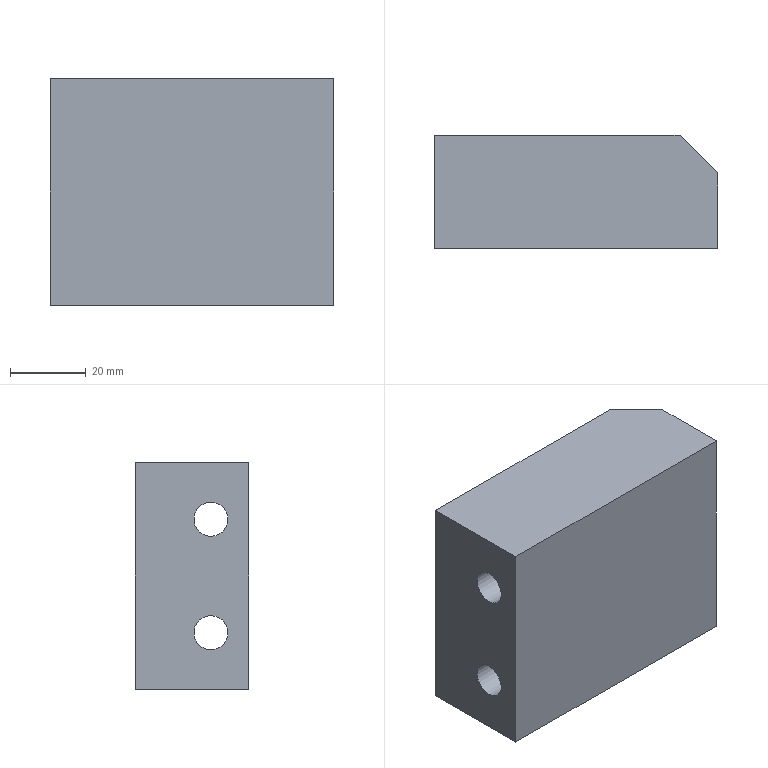Component | NX | BLOCK | 1 solid | 13 faces | box 75 x 30 x 60 mm | volume 109112 mm3 | plane 9 | cylinder 4 | commonest cylinder face diameters 9 x2 15 x2
STEP:
#1=CARTESIAN_POINT('',(0.,0.,0.));
#2=DIRECTION('',(0.,0.,1.));
#3=DIRECTION('',(1.,0.,0.));
#4=AXIS2_PLACEMENT_3D('',#1,#2,#3);
#5=CARTESIAN_POINT('',(2.092,116.121,56.345));
#6=VERTEX_POINT('',#5);
#7=CARTESIAN_POINT('',(2.092,116.121,48.845));
#8=DIRECTION('',(-1.,0.,0.));
#9=DIRECTION('',(0.,0.,1.));
#10=AXIS2_PLACEMENT_3D('',#7,#8,#9);
#11=CIRCLE('',#10,7.5);
#12=CARTESIAN_POINT('',(2.092,121.121,63.845));
#13=DIRECTION('',(1.,0.,0.));
#14=DIRECTION('',(0.,0.,-1.));
#15=AXIS2_PLACEMENT_3D('',#12,#13,#14);
#16=PLANE('',#15);
#17=CARTESIAN_POINT('',(7.5,-5.));
#18=CARTESIAN_POINT('',(7.5,7.99));
#19=CARTESIAN_POINT('',(18.75,1.495));
#20=CARTESIAN_POINT('',(30.,-5.));
#21=CARTESIAN_POINT('',(18.75,-11.495));
#22=CARTESIAN_POINT('',(7.5,-17.99));
#23=CARTESIAN_POINT('',(7.5,-5.));
#24=(BOUNDED_CURVE()B_SPLINE_CURVE(2,(#17,#18,#19,#20,#21,#22,#23),.UNSPECIFIED.,.T.,.F.)B_SPLINE_CURVE_WITH_KNOTS((1,2,2,2,2,1),(-2.094,0.,2.094,4.189,6.283,8.378),.UNSPECIFIED.)CURVE()GEOMETRIC_REPRESENTATION_ITEM()RATIONAL_B_SPLINE_CURVE((1.,0.5,1.,0.5,1.,0.5,1.))REPRESENTATION_ITEM(''));
#25=(GEOMETRIC_REPRESENTATION_CONTEXT(2)PARAMETRIC_REPRESENTATION_CONTEXT()REPRESENTATION_CONTEXT('',''));
#26=DEFINITIONAL_REPRESENTATION('',(#24),#25);
#27=PCURVE('',#16,#26);
#28=CARTESIAN_POINT('',(2.092,116.121,48.845));
#29=DIRECTION('',(-1.,0.,0.));
#30=DIRECTION('',(0.,0.,1.));
#31=AXIS2_PLACEMENT_3D('',#28,#29,#30);
#32=CYLINDRICAL_SURFACE('',#31,7.5);
#33=CARTESIAN_POINT('',(0.,0.));
#34=DIRECTION('',(1.,0.));
#35=VECTOR('',#34,1.);
#36=LINE('',#33,#35);
#37=(GEOMETRIC_REPRESENTATION_CONTEXT(2)PARAMETRIC_REPRESENTATION_CONTEXT()REPRESENTATION_CONTEXT('',''));
#38=DEFINITIONAL_REPRESENTATION('',(#36),#37);
#39=PCURVE('',#32,#38);
#40=SURFACE_CURVE('',#11,(#27,#39),.PCURVE_S1.);
#41=EDGE_CURVE('',#6,#6,#40,.T.);
#42=ORIENTED_EDGE('',*,*,#41,.T.);
#43=EDGE_LOOP('',(#42));
#44=FACE_BOUND('',#43,.T.);
#45=CARTESIAN_POINT('',(2.092,116.121,86.345));
#46=VERTEX_POINT('',#45);
#47=CARTESIAN_POINT('',(2.092,116.121,78.845));
#48=DIRECTION('',(-1.,0.,0.));
#49=DIRECTION('',(0.,0.,1.));
#50=AXIS2_PLACEMENT_3D('',#47,#48,#49);
#51=CIRCLE('',#50,7.5);
#52=CARTESIAN_POINT('',(-22.5,-5.));
#53=CARTESIAN_POINT('',(-22.5,7.99));
#54=CARTESIAN_POINT('',(-11.25,1.495));
#55=CARTESIAN_POINT('',(-0.,-5.));
#56=CARTESIAN_POINT('',(-11.25,-11.495));
#57=CARTESIAN_POINT('',(-22.5,-17.99));
#58=CARTESIAN_POINT('',(-22.5,-5.));
#59=(BOUNDED_CURVE()B_SPLINE_CURVE(2,(#52,#53,#54,#55,#56,#57,#58),.UNSPECIFIED.,.T.,.F.)B_SPLINE_CURVE_WITH_KNOTS((1,2,2,2,2,1),(-2.094,0.,2.094,4.189,6.283,8.378),.UNSPECIFIED.)CURVE()GEOMETRIC_REPRESENTATION_ITEM()RATIONAL_B_SPLINE_CURVE((1.,0.5,1.,0.5,1.,0.5,1.))REPRESENTATION_ITEM(''));
#60=(GEOMETRIC_REPRESENTATION_CONTEXT(2)PARAMETRIC_REPRESENTATION_CONTEXT()REPRESENTATION_CONTEXT('',''));
#61=DEFINITIONAL_REPRESENTATION('',(#59),#60);
#62=PCURVE('',#16,#61);
#63=CARTESIAN_POINT('',(2.092,116.121,78.845));
#64=DIRECTION('',(-1.,0.,0.));
#65=DIRECTION('',(0.,0.,1.));
#66=AXIS2_PLACEMENT_3D('',#63,#64,#65);
#67=CYLINDRICAL_SURFACE('',#66,7.5);
#68=CARTESIAN_POINT('',(0.,0.));
#69=DIRECTION('',(1.,0.));
#70=VECTOR('',#69,1.);
#71=LINE('',#68,#70);
#72=(GEOMETRIC_REPRESENTATION_CONTEXT(2)PARAMETRIC_REPRESENTATION_CONTEXT()REPRESENTATION_CONTEXT('',''));
#73=DEFINITIONAL_REPRESENTATION('',(#71),#72);
#74=PCURVE('',#67,#73);
#75=SURFACE_CURVE('',#51,(#62,#74),.PCURVE_S1.);
#76=EDGE_CURVE('',#46,#46,#75,.T.);
#77=ORIENTED_EDGE('',*,*,#76,.T.);
#78=EDGE_LOOP('',(#77));
#79=FACE_BOUND('',#78,.T.);
#80=CARTESIAN_POINT('',(2.092,126.121,33.845));
#81=VERTEX_POINT('',#80);
#82=CARTESIAN_POINT('',(2.092,106.121,33.845));
#83=VERTEX_POINT('',#82);
#84=CARTESIAN_POINT('',(2.092,121.121,33.845));
#85=DIRECTION('',(0.,-1.,0.));
#86=VECTOR('',#85,1.);
#87=LINE('',#84,#86);
#88=CARTESIAN_POINT('',(30.,0.));
#89=DIRECTION('',(0.,-1.));
#90=VECTOR('',#89,1.);
#91=LINE('',#88,#90);
#92=(GEOMETRIC_REPRESENTATION_CONTEXT(2)PARAMETRIC_REPRESENTATION_CONTEXT()REPRESENTATION_CONTEXT('',''));
#93=DEFINITIONAL_REPRESENTATION('',(#91),#92);
#94=PCURVE('',#16,#93);
#95=CARTESIAN_POINT('',(-72.908,121.121,33.845));
#96=DIRECTION('',(0.,0.,-1.));
#97=DIRECTION('',(-1.,0.,0.));
#98=AXIS2_PLACEMENT_3D('',#95,#96,#97);
#99=PLANE('',#98);
#100=CARTESIAN_POINT('',(-75.,0.));
#101=DIRECTION('',(0.,-1.));
#102=VECTOR('',#101,1.);
#103=LINE('',#100,#102);
#104=(GEOMETRIC_REPRESENTATION_CONTEXT(2)PARAMETRIC_REPRESENTATION_CONTEXT()REPRESENTATION_CONTEXT('',''));
#105=DEFINITIONAL_REPRESENTATION('',(#103),#104);
#106=PCURVE('',#99,#105);
#107=SURFACE_CURVE('',#87,(#94,#106),.PCURVE_S1.);
#108=EDGE_CURVE('',#81,#83,#107,.T.);
#109=ORIENTED_EDGE('',*,*,#108,.F.);
#110=CARTESIAN_POINT('',(2.092,126.121,93.845));
#111=VERTEX_POINT('',#110);
#112=CARTESIAN_POINT('',(2.092,126.121,63.845));
#113=DIRECTION('',(0.,0.,1.));
#114=VECTOR('',#113,1.);
#115=LINE('',#112,#114);
#116=CARTESIAN_POINT('',(0.,5.));
#117=DIRECTION('',(-1.,0.));
#118=VECTOR('',#117,1.);
#119=LINE('',#116,#118);
#120=(GEOMETRIC_REPRESENTATION_CONTEXT(2)PARAMETRIC_REPRESENTATION_CONTEXT()REPRESENTATION_CONTEXT('',''));
#121=DEFINITIONAL_REPRESENTATION('',(#119),#120);
#122=PCURVE('',#16,#121);
#123=CARTESIAN_POINT('',(-7.908,136.121,63.845));
#124=DIRECTION('',(-0.7071,-0.7071,0.));
#125=DIRECTION('',(0.,0.,-1.));
#126=AXIS2_PLACEMENT_3D('',#123,#124,#125);
#127=PLANE('',#126);
#128=CARTESIAN_POINT('',(0.,14.142));
#129=DIRECTION('',(-1.,0.));
#130=VECTOR('',#129,1.);
#131=LINE('',#128,#130);
#132=(GEOMETRIC_REPRESENTATION_CONTEXT(2)PARAMETRIC_REPRESENTATION_CONTEXT()REPRESENTATION_CONTEXT('',''));
#133=DEFINITIONAL_REPRESENTATION('',(#131),#132);
#134=PCURVE('',#127,#133);
#135=SURFACE_CURVE('',#115,(#122,#134),.PCURVE_S1.);
#136=EDGE_CURVE('',#81,#111,#135,.T.);
#137=ORIENTED_EDGE('',*,*,#136,.T.);
#138=CARTESIAN_POINT('',(2.092,106.121,93.845));
#139=VERTEX_POINT('',#138);
#140=CARTESIAN_POINT('',(2.092,121.121,93.845));
#141=DIRECTION('',(0.,1.,0.));
#142=VECTOR('',#141,1.);
#143=LINE('',#140,#142);
#144=CARTESIAN_POINT('',(-30.,0.));
#145=DIRECTION('',(0.,1.));
#146=VECTOR('',#145,1.);
#147=LINE('',#144,#146);
#148=(GEOMETRIC_REPRESENTATION_CONTEXT(2)PARAMETRIC_REPRESENTATION_CONTEXT()REPRESENTATION_CONTEXT('',''));
#149=DEFINITIONAL_REPRESENTATION('',(#147),#148);
#150=PCURVE('',#16,#149);
#151=CARTESIAN_POINT('',(-72.908,121.121,93.845));
#152=DIRECTION('',(0.,0.,1.));
#153=DIRECTION('',(1.,0.,0.));
#154=AXIS2_PLACEMENT_3D('',#151,#152,#153);
#155=PLANE('',#154);
#156=CARTESIAN_POINT('',(75.,0.));
#157=DIRECTION('',(0.,1.));
#158=VECTOR('',#157,1.);
#159=LINE('',#156,#158);
#160=(GEOMETRIC_REPRESENTATION_CONTEXT(2)PARAMETRIC_REPRESENTATION_CONTEXT()REPRESENTATION_CONTEXT('',''));
#161=DEFINITIONAL_REPRESENTATION('',(#159),#160);
#162=PCURVE('',#155,#161);
#163=SURFACE_CURVE('',#143,(#150,#162),.PCURVE_S1.);
#164=EDGE_CURVE('',#139,#111,#163,.T.);
#165=ORIENTED_EDGE('',*,*,#164,.F.);
#166=CARTESIAN_POINT('',(2.092,106.121,63.845));
#167=DIRECTION('',(0.,0.,1.));
#168=VECTOR('',#167,1.);
#169=LINE('',#166,#168);
#170=CARTESIAN_POINT('',(0.,-15.));
#171=DIRECTION('',(-1.,0.));
#172=VECTOR('',#171,1.);
#173=LINE('',#170,#172);
#174=(GEOMETRIC_REPRESENTATION_CONTEXT(2)PARAMETRIC_REPRESENTATION_CONTEXT()REPRESENTATION_CONTEXT('',''));
#175=DEFINITIONAL_REPRESENTATION('',(#173),#174);
#176=PCURVE('',#16,#175);
#177=CARTESIAN_POINT('',(-72.908,106.121,63.845));
#178=DIRECTION('',(0.,-1.,0.));
#179=DIRECTION('',(-1.,0.,0.));
#180=AXIS2_PLACEMENT_3D('',#177,#178,#179);
#181=PLANE('',#180);
#182=CARTESIAN_POINT('',(-75.,0.));
#183=DIRECTION('',(0.,-1.));
#184=VECTOR('',#183,1.);
#185=LINE('',#182,#184);
#186=(GEOMETRIC_REPRESENTATION_CONTEXT(2)PARAMETRIC_REPRESENTATION_CONTEXT()REPRESENTATION_CONTEXT('',''));
#187=DEFINITIONAL_REPRESENTATION('',(#185),#186);
#188=PCURVE('',#181,#187);
#189=SURFACE_CURVE('',#169,(#176,#188),.PCURVE_S1.);
#190=EDGE_CURVE('',#83,#139,#189,.T.);
#191=ORIENTED_EDGE('',*,*,#190,.F.);
#192=EDGE_LOOP('',(#109,#137,#165,#191));
#193=FACE_BOUND('',#192,.T.);
#194=ADVANCED_FACE('',(#44,#79,#193),#16,.T.);
#195=CARTESIAN_POINT('',(-72.908,106.121,33.845));
#196=VERTEX_POINT('',#195);
#197=CARTESIAN_POINT('',(-72.908,106.121,33.845));
#198=DIRECTION('',(1.,0.,0.));
#199=VECTOR('',#198,1.);
#200=LINE('',#197,#199);
#201=CARTESIAN_POINT('',(0.,30.));
#202=DIRECTION('',(-1.,0.));
#203=VECTOR('',#202,1.);
#204=LINE('',#201,#203);
#205=(GEOMETRIC_REPRESENTATION_CONTEXT(2)PARAMETRIC_REPRESENTATION_CONTEXT()REPRESENTATION_CONTEXT('',''));
#206=DEFINITIONAL_REPRESENTATION('',(#204),#205);
#207=PCURVE('',#181,#206);
#208=CARTESIAN_POINT('',(0.,-15.));
#209=DIRECTION('',(-1.,0.));
#210=VECTOR('',#209,1.);
#211=LINE('',#208,#210);
#212=(GEOMETRIC_REPRESENTATION_CONTEXT(2)PARAMETRIC_REPRESENTATION_CONTEXT()REPRESENTATION_CONTEXT('',''));
#213=DEFINITIONAL_REPRESENTATION('',(#211),#212);
#214=PCURVE('',#99,#213);
#215=SURFACE_CURVE('',#200,(#207,#214),.PCURVE_S1.);
#216=EDGE_CURVE('',#196,#83,#215,.T.);
#217=ORIENTED_EDGE('',*,*,#216,.T.);
#218=ORIENTED_EDGE('',*,*,#190,.T.);
#219=CARTESIAN_POINT('',(-72.908,106.121,93.845));
#220=VERTEX_POINT('',#219);
#221=CARTESIAN_POINT('',(-72.908,106.121,93.845));
#222=DIRECTION('',(1.,0.,0.));
#223=VECTOR('',#222,1.);
#224=LINE('',#221,#223);
#225=CARTESIAN_POINT('',(0.,-30.));
#226=DIRECTION('',(-1.,0.));
#227=VECTOR('',#226,1.);
#228=LINE('',#225,#227);
#229=(GEOMETRIC_REPRESENTATION_CONTEXT(2)PARAMETRIC_REPRESENTATION_CONTEXT()REPRESENTATION_CONTEXT('',''));
#230=DEFINITIONAL_REPRESENTATION('',(#228),#229);
#231=PCURVE('',#181,#230);
#232=CARTESIAN_POINT('',(0.,-15.));
#233=DIRECTION('',(1.,0.));
#234=VECTOR('',#233,1.);
#235=LINE('',#232,#234);
#236=(GEOMETRIC_REPRESENTATION_CONTEXT(2)PARAMETRIC_REPRESENTATION_CONTEXT()REPRESENTATION_CONTEXT('',''));
#237=DEFINITIONAL_REPRESENTATION('',(#235),#236);
#238=PCURVE('',#155,#237);
#239=SURFACE_CURVE('',#224,(#231,#238),.PCURVE_S1.);
#240=EDGE_CURVE('',#220,#139,#239,.T.);
#241=ORIENTED_EDGE('',*,*,#240,.F.);
#242=CARTESIAN_POINT('',(-72.908,106.121,63.845));
#243=DIRECTION('',(0.,0.,-1.));
#244=VECTOR('',#243,1.);
#245=LINE('',#242,#244);
#246=CARTESIAN_POINT('',(0.,0.));
#247=DIRECTION('',(0.,1.));
#248=VECTOR('',#247,1.);
#249=LINE('',#246,#248);
#250=(GEOMETRIC_REPRESENTATION_CONTEXT(2)PARAMETRIC_REPRESENTATION_CONTEXT()REPRESENTATION_CONTEXT('',''));
#251=DEFINITIONAL_REPRESENTATION('',(#249),#250);
#252=PCURVE('',#181,#251);
#253=CARTESIAN_POINT('',(-72.908,121.121,63.845));
#254=DIRECTION('',(-1.,0.,0.));
#255=DIRECTION('',(0.,0.,1.));
#256=AXIS2_PLACEMENT_3D('',#253,#254,#255);
#257=PLANE('',#256);
#258=CARTESIAN_POINT('',(0.,-15.));
#259=DIRECTION('',(-1.,0.));
#260=VECTOR('',#259,1.);
#261=LINE('',#258,#260);
#262=(GEOMETRIC_REPRESENTATION_CONTEXT(2)PARAMETRIC_REPRESENTATION_CONTEXT()REPRESENTATION_CONTEXT('',''));
#263=DEFINITIONAL_REPRESENTATION('',(#261),#262);
#264=PCURVE('',#257,#263);
#265=SURFACE_CURVE('',#245,(#252,#264),.PCURVE_S1.);
#266=EDGE_CURVE('',#220,#196,#265,.T.);
#267=ORIENTED_EDGE('',*,*,#266,.T.);
#268=EDGE_LOOP('',(#217,#218,#241,#267));
#269=FACE_BOUND('',#268,.T.);
#270=ADVANCED_FACE('',(#269),#181,.T.);
#271=ORIENTED_EDGE('',*,*,#164,.T.);
#272=CARTESIAN_POINT('',(-7.908,136.121,93.845));
#273=VERTEX_POINT('',#272);
#274=CARTESIAN_POINT('',(-32.908,161.121,93.845));
#275=DIRECTION('',(-0.7071,0.7071,0.));
#276=VECTOR('',#275,1.);
#277=LINE('',#274,#276);
#278=CARTESIAN_POINT('',(40.,40.));
#279=DIRECTION('',(-0.7071,0.7071));
#280=VECTOR('',#279,1.);
#281=LINE('',#278,#280);
#282=(GEOMETRIC_REPRESENTATION_CONTEXT(2)PARAMETRIC_REPRESENTATION_CONTEXT()REPRESENTATION_CONTEXT('',''));
#283=DEFINITIONAL_REPRESENTATION('',(#281),#282);
#284=PCURVE('',#155,#283);
#285=CARTESIAN_POINT('',(-30.,-35.355));
#286=DIRECTION('',(0.,-1.));
#287=VECTOR('',#286,1.);
#288=LINE('',#285,#287);
#289=(GEOMETRIC_REPRESENTATION_CONTEXT(2)PARAMETRIC_REPRESENTATION_CONTEXT()REPRESENTATION_CONTEXT('',''));
#290=DEFINITIONAL_REPRESENTATION('',(#288),#289);
#291=PCURVE('',#127,#290);
#292=SURFACE_CURVE('',#277,(#284,#291),.PCURVE_S1.);
#293=EDGE_CURVE('',#111,#273,#292,.T.);
#294=ORIENTED_EDGE('',*,*,#293,.T.);
#295=CARTESIAN_POINT('',(-72.908,136.121,93.845));
#296=VERTEX_POINT('',#295);
#297=CARTESIAN_POINT('',(-72.908,136.121,93.845));
#298=DIRECTION('',(1.,0.,0.));
#299=VECTOR('',#298,1.);
#300=LINE('',#297,#299);
#301=CARTESIAN_POINT('',(0.,15.));
#302=DIRECTION('',(1.,0.));
#303=VECTOR('',#302,1.);
#304=LINE('',#301,#303);
#305=(GEOMETRIC_REPRESENTATION_CONTEXT(2)PARAMETRIC_REPRESENTATION_CONTEXT()REPRESENTATION_CONTEXT('',''));
#306=DEFINITIONAL_REPRESENTATION('',(#304),#305);
#307=PCURVE('',#155,#306);
#308=CARTESIAN_POINT('',(-72.908,136.121,63.845));
#309=DIRECTION('',(0.,1.,0.));
#310=DIRECTION('',(1.,0.,0.));
#311=AXIS2_PLACEMENT_3D('',#308,#309,#310);
#312=PLANE('',#311);
#313=CARTESIAN_POINT('',(0.,-30.));
#314=DIRECTION('',(1.,0.));
#315=VECTOR('',#314,1.);
#316=LINE('',#313,#315);
#317=(GEOMETRIC_REPRESENTATION_CONTEXT(2)PARAMETRIC_REPRESENTATION_CONTEXT()REPRESENTATION_CONTEXT('',''));
#318=DEFINITIONAL_REPRESENTATION('',(#316),#317);
#319=PCURVE('',#312,#318);
#320=SURFACE_CURVE('',#300,(#307,#319),.PCURVE_S1.);
#321=EDGE_CURVE('',#296,#273,#320,.T.);
#322=ORIENTED_EDGE('',*,*,#321,.F.);
#323=CARTESIAN_POINT('',(-72.908,121.121,93.845));
#324=DIRECTION('',(0.,-1.,0.));
#325=VECTOR('',#324,1.);
#326=LINE('',#323,#325);
#327=CARTESIAN_POINT('',(0.,0.));
#328=DIRECTION('',(0.,-1.));
#329=VECTOR('',#328,1.);
#330=LINE('',#327,#329);
#331=(GEOMETRIC_REPRESENTATION_CONTEXT(2)PARAMETRIC_REPRESENTATION_CONTEXT()REPRESENTATION_CONTEXT('',''));
#332=DEFINITIONAL_REPRESENTATION('',(#330),#331);
#333=PCURVE('',#155,#332);
#334=CARTESIAN_POINT('',(30.,0.));
#335=DIRECTION('',(0.,-1.));
#336=VECTOR('',#335,1.);
#337=LINE('',#334,#336);
#338=(GEOMETRIC_REPRESENTATION_CONTEXT(2)PARAMETRIC_REPRESENTATION_CONTEXT()REPRESENTATION_CONTEXT('',''));
#339=DEFINITIONAL_REPRESENTATION('',(#337),#338);
#340=PCURVE('',#257,#339);
#341=SURFACE_CURVE('',#326,(#333,#340),.PCURVE_S1.);
#342=EDGE_CURVE('',#296,#220,#341,.T.);
#343=ORIENTED_EDGE('',*,*,#342,.T.);
#344=ORIENTED_EDGE('',*,*,#240,.T.);
#345=EDGE_LOOP('',(#271,#294,#322,#343,#344));
#346=FACE_BOUND('',#345,.T.);
#347=ADVANCED_FACE('',(#346),#155,.T.);
#348=ORIENTED_EDGE('',*,*,#321,.T.);
#349=CARTESIAN_POINT('',(-7.908,136.121,33.845));
#350=VERTEX_POINT('',#349);
#351=CARTESIAN_POINT('',(-7.908,136.121,63.845));
#352=DIRECTION('',(0.,0.,-1.));
#353=VECTOR('',#352,1.);
#354=LINE('',#351,#353);
#355=CARTESIAN_POINT('',(65.,0.));
#356=DIRECTION('',(0.,1.));
#357=VECTOR('',#356,1.);
#358=LINE('',#355,#357);
#359=(GEOMETRIC_REPRESENTATION_CONTEXT(2)PARAMETRIC_REPRESENTATION_CONTEXT()REPRESENTATION_CONTEXT('',''));
#360=DEFINITIONAL_REPRESENTATION('',(#358),#359);
#361=PCURVE('',#312,#360);
#362=CARTESIAN_POINT('',(0.,0.));
#363=DIRECTION('',(1.,0.));
#364=VECTOR('',#363,1.);
#365=LINE('',#362,#364);
#366=(GEOMETRIC_REPRESENTATION_CONTEXT(2)PARAMETRIC_REPRESENTATION_CONTEXT()REPRESENTATION_CONTEXT('',''));
#367=DEFINITIONAL_REPRESENTATION('',(#365),#366);
#368=PCURVE('',#127,#367);
#369=SURFACE_CURVE('',#354,(#361,#368),.PCURVE_S1.);
#370=EDGE_CURVE('',#273,#350,#369,.T.);
#371=ORIENTED_EDGE('',*,*,#370,.T.);
#372=CARTESIAN_POINT('',(-72.908,136.121,33.845));
#373=VERTEX_POINT('',#372);
#374=CARTESIAN_POINT('',(-72.908,136.121,33.845));
#375=DIRECTION('',(1.,0.,0.));
#376=VECTOR('',#375,1.);
#377=LINE('',#374,#376);
#378=CARTESIAN_POINT('',(0.,30.));
#379=DIRECTION('',(1.,0.));
#380=VECTOR('',#379,1.);
#381=LINE('',#378,#380);
#382=(GEOMETRIC_REPRESENTATION_CONTEXT(2)PARAMETRIC_REPRESENTATION_CONTEXT()REPRESENTATION_CONTEXT('',''));
#383=DEFINITIONAL_REPRESENTATION('',(#381),#382);
#384=PCURVE('',#312,#383);
#385=CARTESIAN_POINT('',(0.,15.));
#386=DIRECTION('',(-1.,0.));
#387=VECTOR('',#386,1.);
#388=LINE('',#385,#387);
#389=(GEOMETRIC_REPRESENTATION_CONTEXT(2)PARAMETRIC_REPRESENTATION_CONTEXT()REPRESENTATION_CONTEXT('',''));
#390=DEFINITIONAL_REPRESENTATION('',(#388),#389);
#391=PCURVE('',#99,#390);
#392=SURFACE_CURVE('',#377,(#384,#391),.PCURVE_S1.);
#393=EDGE_CURVE('',#373,#350,#392,.T.);
#394=ORIENTED_EDGE('',*,*,#393,.F.);
#395=CARTESIAN_POINT('',(-72.908,136.121,63.845));
#396=DIRECTION('',(0.,0.,1.));
#397=VECTOR('',#396,1.);
#398=LINE('',#395,#397);
#399=CARTESIAN_POINT('',(0.,0.));
#400=DIRECTION('',(0.,-1.));
#401=VECTOR('',#400,1.);
#402=LINE('',#399,#401);
#403=(GEOMETRIC_REPRESENTATION_CONTEXT(2)PARAMETRIC_REPRESENTATION_CONTEXT()REPRESENTATION_CONTEXT('',''));
#404=DEFINITIONAL_REPRESENTATION('',(#402),#403);
#405=PCURVE('',#312,#404);
#406=CARTESIAN_POINT('',(0.,15.));
#407=DIRECTION('',(1.,0.));
#408=VECTOR('',#407,1.);
#409=LINE('',#406,#408);
#410=(GEOMETRIC_REPRESENTATION_CONTEXT(2)PARAMETRIC_REPRESENTATION_CONTEXT()REPRESENTATION_CONTEXT('',''));
#411=DEFINITIONAL_REPRESENTATION('',(#409),#410);
#412=PCURVE('',#257,#411);
#413=SURFACE_CURVE('',#398,(#405,#412),.PCURVE_S1.);
#414=EDGE_CURVE('',#373,#296,#413,.T.);
#415=ORIENTED_EDGE('',*,*,#414,.T.);
#416=EDGE_LOOP('',(#348,#371,#394,#415));
#417=FACE_BOUND('',#416,.T.);
#418=ADVANCED_FACE('',(#417),#312,.T.);
#419=CARTESIAN_POINT('',(-72.908,116.121,53.345));
#420=VERTEX_POINT('',#419);
#421=CARTESIAN_POINT('',(-72.908,116.121,48.845));
#422=DIRECTION('',(-1.,0.,0.));
#423=DIRECTION('',(0.,0.,1.));
#424=AXIS2_PLACEMENT_3D('',#421,#422,#423);
#425=CIRCLE('',#424,4.5);
#426=CARTESIAN_POINT('',(-15.,-5.));
#427=DIRECTION('',(1.,0.));
#428=AXIS2_PLACEMENT_2D('',#426,#427);
#429=CIRCLE('',#428,4.5);
#430=(GEOMETRIC_REPRESENTATION_CONTEXT(2)PARAMETRIC_REPRESENTATION_CONTEXT()REPRESENTATION_CONTEXT('',''));
#431=DEFINITIONAL_REPRESENTATION('',(#429),#430);
#432=PCURVE('',#257,#431);
#433=CARTESIAN_POINT('',(-88.444,116.121,48.845));
#434=DIRECTION('',(-1.,0.,0.));
#435=DIRECTION('',(0.,0.,1.));
#436=AXIS2_PLACEMENT_3D('',#433,#434,#435);
#437=CYLINDRICAL_SURFACE('',#436,4.5);
#438=CARTESIAN_POINT('',(0.,-15.536));
#439=DIRECTION('',(1.,0.));
#440=VECTOR('',#439,1.);
#441=LINE('',#438,#440);
#442=(GEOMETRIC_REPRESENTATION_CONTEXT(2)PARAMETRIC_REPRESENTATION_CONTEXT()REPRESENTATION_CONTEXT('',''));
#443=DEFINITIONAL_REPRESENTATION('',(#441),#442);
#444=PCURVE('',#437,#443);
#445=SURFACE_CURVE('',#425,(#432,#444),.PCURVE_S1.);
#446=EDGE_CURVE('',#420,#420,#445,.T.);
#447=ORIENTED_EDGE('',*,*,#446,.F.);
#448=EDGE_LOOP('',(#447));
#449=FACE_BOUND('',#448,.T.);
#450=CARTESIAN_POINT('',(-72.908,116.121,83.345));
#451=VERTEX_POINT('',#450);
#452=CARTESIAN_POINT('',(-72.908,116.121,78.845));
#453=DIRECTION('',(-1.,0.,0.));
#454=DIRECTION('',(0.,0.,1.));
#455=AXIS2_PLACEMENT_3D('',#452,#453,#454);
#456=CIRCLE('',#455,4.5);
#457=CARTESIAN_POINT('',(15.,-5.));
#458=DIRECTION('',(1.,0.));
#459=AXIS2_PLACEMENT_2D('',#457,#458);
#460=CIRCLE('',#459,4.5);
#461=(GEOMETRIC_REPRESENTATION_CONTEXT(2)PARAMETRIC_REPRESENTATION_CONTEXT()REPRESENTATION_CONTEXT('',''));
#462=DEFINITIONAL_REPRESENTATION('',(#460),#461);
#463=PCURVE('',#257,#462);
#464=CARTESIAN_POINT('',(-88.444,116.121,78.845));
#465=DIRECTION('',(-1.,0.,0.));
#466=DIRECTION('',(0.,0.,1.));
#467=AXIS2_PLACEMENT_3D('',#464,#465,#466);
#468=CYLINDRICAL_SURFACE('',#467,4.5);
#469=CARTESIAN_POINT('',(0.,-15.536));
#470=DIRECTION('',(1.,0.));
#471=VECTOR('',#470,1.);
#472=LINE('',#469,#471);
#473=(GEOMETRIC_REPRESENTATION_CONTEXT(2)PARAMETRIC_REPRESENTATION_CONTEXT()REPRESENTATION_CONTEXT('',''));
#474=DEFINITIONAL_REPRESENTATION('',(#472),#473);
#475=PCURVE('',#468,#474);
#476=SURFACE_CURVE('',#456,(#463,#475),.PCURVE_S1.);
#477=EDGE_CURVE('',#451,#451,#476,.T.);
#478=ORIENTED_EDGE('',*,*,#477,.F.);
#479=EDGE_LOOP('',(#478));
#480=FACE_BOUND('',#479,.T.);
#481=CARTESIAN_POINT('',(-72.908,121.121,33.845));
#482=DIRECTION('',(0.,1.,0.));
#483=VECTOR('',#482,1.);
#484=LINE('',#481,#483);
#485=CARTESIAN_POINT('',(-30.,0.));
#486=DIRECTION('',(0.,1.));
#487=VECTOR('',#486,1.);
#488=LINE('',#485,#487);
#489=(GEOMETRIC_REPRESENTATION_CONTEXT(2)PARAMETRIC_REPRESENTATION_CONTEXT()REPRESENTATION_CONTEXT('',''));
#490=DEFINITIONAL_REPRESENTATION('',(#488),#489);
#491=PCURVE('',#257,#490);
#492=CARTESIAN_POINT('',(0.,0.));
#493=DIRECTION('',(0.,1.));
#494=VECTOR('',#493,1.);
#495=LINE('',#492,#494);
#496=(GEOMETRIC_REPRESENTATION_CONTEXT(2)PARAMETRIC_REPRESENTATION_CONTEXT()REPRESENTATION_CONTEXT('',''));
#497=DEFINITIONAL_REPRESENTATION('',(#495),#496);
#498=PCURVE('',#99,#497);
#499=SURFACE_CURVE('',#484,(#491,#498),.PCURVE_S1.);
#500=EDGE_CURVE('',#196,#373,#499,.T.);
#501=ORIENTED_EDGE('',*,*,#500,.F.);
#502=ORIENTED_EDGE('',*,*,#266,.F.);
#503=ORIENTED_EDGE('',*,*,#342,.F.);
#504=ORIENTED_EDGE('',*,*,#414,.F.);
#505=EDGE_LOOP('',(#501,#502,#503,#504));
#506=FACE_BOUND('',#505,.T.);
#507=ADVANCED_FACE('',(#449,#480,#506),#257,.T.);
#508=ORIENTED_EDGE('',*,*,#393,.T.);
#509=CARTESIAN_POINT('',(-32.908,161.121,33.845));
#510=DIRECTION('',(0.7071,-0.7071,0.));
#511=VECTOR('',#510,1.);
#512=LINE('',#509,#511);
#513=CARTESIAN_POINT('',(-40.,40.));
#514=DIRECTION('',(-0.7071,-0.7071));
#515=VECTOR('',#514,1.);
#516=LINE('',#513,#515);
#517=(GEOMETRIC_REPRESENTATION_CONTEXT(2)PARAMETRIC_REPRESENTATION_CONTEXT()REPRESENTATION_CONTEXT('',''));
#518=DEFINITIONAL_REPRESENTATION('',(#516),#517);
#519=PCURVE('',#99,#518);
#520=CARTESIAN_POINT('',(30.,-35.355));
#521=DIRECTION('',(0.,1.));
#522=VECTOR('',#521,1.);
#523=LINE('',#520,#522);
#524=(GEOMETRIC_REPRESENTATION_CONTEXT(2)PARAMETRIC_REPRESENTATION_CONTEXT()REPRESENTATION_CONTEXT('',''));
#525=DEFINITIONAL_REPRESENTATION('',(#523),#524);
#526=PCURVE('',#127,#525);
#527=SURFACE_CURVE('',#512,(#519,#526),.PCURVE_S1.);
#528=EDGE_CURVE('',#350,#81,#527,.T.);
#529=ORIENTED_EDGE('',*,*,#528,.T.);
#530=ORIENTED_EDGE('',*,*,#108,.T.);
#531=ORIENTED_EDGE('',*,*,#216,.F.);
#532=ORIENTED_EDGE('',*,*,#500,.T.);
#533=EDGE_LOOP('',(#508,#529,#530,#531,#532));
#534=FACE_BOUND('',#533,.T.);
#535=ADVANCED_FACE('',(#534),#99,.T.);
#536=ORIENTED_EDGE('',*,*,#293,.F.);
#537=ORIENTED_EDGE('',*,*,#136,.F.);
#538=ORIENTED_EDGE('',*,*,#528,.F.);
#539=ORIENTED_EDGE('',*,*,#370,.F.);
#540=EDGE_LOOP('',(#536,#537,#538,#539));
#541=FACE_BOUND('',#540,.T.);
#542=ADVANCED_FACE('',(#541),#127,.F.);
#543=ORIENTED_EDGE('',*,*,#477,.F.);
#544=CARTESIAN_POINT('',(-56.908,116.121,83.345));
#545=VERTEX_POINT('',#544);
#546=CARTESIAN_POINT('',(-56.908,116.121,83.345));
#547=CARTESIAN_POINT('',(-72.908,116.121,83.345));
#548=B_SPLINE_CURVE_WITH_KNOTS('',1,(#546,#547),.UNSPECIFIED.,.F.,.F.,(2,2),(-31.536,-15.536),.PIECEWISE_BEZIER_KNOTS.);
#549=CARTESIAN_POINT('',(0.,0.));
#550=DIRECTION('',(0.,1.));
#551=VECTOR('',#550,1.);
#552=LINE('',#549,#551);
#553=(GEOMETRIC_REPRESENTATION_CONTEXT(2)PARAMETRIC_REPRESENTATION_CONTEXT()REPRESENTATION_CONTEXT('',''));
#554=DEFINITIONAL_REPRESENTATION('',(#552),#553);
#555=PCURVE('',#468,#554);
#556=CARTESIAN_POINT('',(6.283,0.));
#557=DIRECTION('',(0.,1.));
#558=VECTOR('',#557,1.);
#559=LINE('',#556,#558);
#560=(GEOMETRIC_REPRESENTATION_CONTEXT(2)PARAMETRIC_REPRESENTATION_CONTEXT()REPRESENTATION_CONTEXT('',''));
#561=DEFINITIONAL_REPRESENTATION('',(#559),#560);
#562=PCURVE('',#468,#561);
#563=SEAM_CURVE('',#548,(#555,#562),.PCURVE_S1.);
#564=EDGE_CURVE('',#545,#451,#563,.T.);
#565=ORIENTED_EDGE('',*,*,#564,.F.);
#566=CARTESIAN_POINT('',(-56.908,116.121,78.845));
#567=DIRECTION('',(1.,0.,0.));
#568=DIRECTION('',(0.,0.,1.));
#569=AXIS2_PLACEMENT_3D('',#566,#567,#568);
#570=CIRCLE('',#569,4.5);
#571=CARTESIAN_POINT('',(6.283,-31.536));
#572=DIRECTION('',(-1.,0.));
#573=VECTOR('',#572,1.);
#574=LINE('',#571,#573);
#575=(GEOMETRIC_REPRESENTATION_CONTEXT(2)PARAMETRIC_REPRESENTATION_CONTEXT()REPRESENTATION_CONTEXT('',''));
#576=DEFINITIONAL_REPRESENTATION('',(#574),#575);
#577=PCURVE('',#468,#576);
#578=CARTESIAN_POINT('',(-56.908,116.121,78.845));
#579=DIRECTION('',(-1.,0.,0.));
#580=DIRECTION('',(0.,0.,1.));
#581=AXIS2_PLACEMENT_3D('',#578,#579,#580);
#582=PLANE('',#581);
#583=CARTESIAN_POINT('',(4.5,0.));
#584=CARTESIAN_POINT('',(4.5,-7.794));
#585=CARTESIAN_POINT('',(-2.25,-3.897));
#586=CARTESIAN_POINT('',(-9.,-0.));
#587=CARTESIAN_POINT('',(-2.25,3.897));
#588=CARTESIAN_POINT('',(4.5,7.794));
#589=CARTESIAN_POINT('',(4.5,0.));
#590=(BOUNDED_CURVE()B_SPLINE_CURVE(2,(#583,#584,#585,#586,#587,#588,#589),.UNSPECIFIED.,.T.,.F.)B_SPLINE_CURVE_WITH_KNOTS((1,2,2,2,2,1),(-2.094,0.,2.094,4.189,6.283,8.378),.UNSPECIFIED.)CURVE()GEOMETRIC_REPRESENTATION_ITEM()RATIONAL_B_SPLINE_CURVE((1.,0.5,1.,0.5,1.,0.5,1.))REPRESENTATION_ITEM(''));
#591=(GEOMETRIC_REPRESENTATION_CONTEXT(2)PARAMETRIC_REPRESENTATION_CONTEXT()REPRESENTATION_CONTEXT('',''));
#592=DEFINITIONAL_REPRESENTATION('',(#590),#591);
#593=PCURVE('',#582,#592);
#594=SURFACE_CURVE('',#570,(#577,#593),.PCURVE_S1.);
#595=EDGE_CURVE('',#545,#545,#594,.T.);
#596=ORIENTED_EDGE('',*,*,#595,.F.);
#597=ORIENTED_EDGE('',*,*,#564,.T.);
#598=EDGE_LOOP('',(#543,#565,#596,#597));
#599=FACE_BOUND('',#598,.F.);
#600=ADVANCED_FACE('',(#599),#468,.F.);
#601=ORIENTED_EDGE('',*,*,#595,.F.);
#602=EDGE_LOOP('',(#601));
#603=FACE_BOUND('',#602,.T.);
#604=CARTESIAN_POINT('',(-56.908,116.121,86.345));
#605=VERTEX_POINT('',#604);
#606=CARTESIAN_POINT('',(-56.908,116.121,78.845));
#607=DIRECTION('',(1.,0.,0.));
#608=DIRECTION('',(0.,0.,1.));
#609=AXIS2_PLACEMENT_3D('',#606,#607,#608);
#610=CIRCLE('',#609,7.5);
#611=CARTESIAN_POINT('',(7.5,0.));
#612=CARTESIAN_POINT('',(7.5,-12.99));
#613=CARTESIAN_POINT('',(-3.75,-6.495));
#614=CARTESIAN_POINT('',(-15.,-0.));
#615=CARTESIAN_POINT('',(-3.75,6.495));
#616=CARTESIAN_POINT('',(7.5,12.99));
#617=CARTESIAN_POINT('',(7.5,0.));
#618=(BOUNDED_CURVE()B_SPLINE_CURVE(2,(#611,#612,#613,#614,#615,#616,#617),.UNSPECIFIED.,.T.,.F.)B_SPLINE_CURVE_WITH_KNOTS((1,2,2,2,2,1),(-2.094,0.,2.094,4.189,6.283,8.378),.UNSPECIFIED.)CURVE()GEOMETRIC_REPRESENTATION_ITEM()RATIONAL_B_SPLINE_CURVE((1.,0.5,1.,0.5,1.,0.5,1.))REPRESENTATION_ITEM(''));
#619=(GEOMETRIC_REPRESENTATION_CONTEXT(2)PARAMETRIC_REPRESENTATION_CONTEXT()REPRESENTATION_CONTEXT('',''));
#620=DEFINITIONAL_REPRESENTATION('',(#618),#619);
#621=PCURVE('',#582,#620);
#622=CARTESIAN_POINT('',(6.283,59.));
#623=DIRECTION('',(-1.,0.));
#624=VECTOR('',#623,1.);
#625=LINE('',#622,#624);
#626=(GEOMETRIC_REPRESENTATION_CONTEXT(2)PARAMETRIC_REPRESENTATION_CONTEXT()REPRESENTATION_CONTEXT('',''));
#627=DEFINITIONAL_REPRESENTATION('',(#625),#626);
#628=PCURVE('',#67,#627);
#629=SURFACE_CURVE('',#610,(#621,#628),.PCURVE_S1.);
#630=EDGE_CURVE('',#605,#605,#629,.T.);
#631=ORIENTED_EDGE('',*,*,#630,.T.);
#632=EDGE_LOOP('',(#631));
#633=FACE_BOUND('',#632,.T.);
#634=ADVANCED_FACE('',(#603,#633),#582,.F.);
#635=ORIENTED_EDGE('',*,*,#630,.T.);
#636=CARTESIAN_POINT('',(2.092,116.121,86.345));
#637=CARTESIAN_POINT('',(-56.908,116.121,86.345));
#638=B_SPLINE_CURVE_WITH_KNOTS('',1,(#636,#637),.UNSPECIFIED.,.F.,.F.,(2,2),(0.,59.),.PIECEWISE_BEZIER_KNOTS.);
#639=CARTESIAN_POINT('',(0.,0.));
#640=DIRECTION('',(0.,1.));
#641=VECTOR('',#640,1.);
#642=LINE('',#639,#641);
#643=(GEOMETRIC_REPRESENTATION_CONTEXT(2)PARAMETRIC_REPRESENTATION_CONTEXT()REPRESENTATION_CONTEXT('',''));
#644=DEFINITIONAL_REPRESENTATION('',(#642),#643);
#645=PCURVE('',#67,#644);
#646=CARTESIAN_POINT('',(6.283,0.));
#647=DIRECTION('',(0.,1.));
#648=VECTOR('',#647,1.);
#649=LINE('',#646,#648);
#650=(GEOMETRIC_REPRESENTATION_CONTEXT(2)PARAMETRIC_REPRESENTATION_CONTEXT()REPRESENTATION_CONTEXT('',''));
#651=DEFINITIONAL_REPRESENTATION('',(#649),#650);
#652=PCURVE('',#67,#651);
#653=SEAM_CURVE('',#638,(#645,#652),.PCURVE_S1.);
#654=EDGE_CURVE('',#46,#605,#653,.T.);
#655=ORIENTED_EDGE('',*,*,#654,.F.);
#656=ORIENTED_EDGE('',*,*,#76,.T.);
#657=ORIENTED_EDGE('',*,*,#654,.T.);
#658=EDGE_LOOP('',(#635,#655,#656,#657));
#659=FACE_BOUND('',#658,.F.);
#660=ADVANCED_FACE('',(#659),#67,.F.);
#661=ORIENTED_EDGE('',*,*,#446,.F.);
#662=CARTESIAN_POINT('',(-56.908,116.121,53.345));
#663=VERTEX_POINT('',#662);
#664=CARTESIAN_POINT('',(-56.908,116.121,53.345));
#665=CARTESIAN_POINT('',(-72.908,116.121,53.345));
#666=B_SPLINE_CURVE_WITH_KNOTS('',1,(#664,#665),.UNSPECIFIED.,.F.,.F.,(2,2),(-31.536,-15.536),.PIECEWISE_BEZIER_KNOTS.);
#667=CARTESIAN_POINT('',(0.,0.));
#668=DIRECTION('',(0.,1.));
#669=VECTOR('',#668,1.);
#670=LINE('',#667,#669);
#671=(GEOMETRIC_REPRESENTATION_CONTEXT(2)PARAMETRIC_REPRESENTATION_CONTEXT()REPRESENTATION_CONTEXT('',''));
#672=DEFINITIONAL_REPRESENTATION('',(#670),#671);
#673=PCURVE('',#437,#672);
#674=CARTESIAN_POINT('',(6.283,0.));
#675=DIRECTION('',(0.,1.));
#676=VECTOR('',#675,1.);
#677=LINE('',#674,#676);
#678=(GEOMETRIC_REPRESENTATION_CONTEXT(2)PARAMETRIC_REPRESENTATION_CONTEXT()REPRESENTATION_CONTEXT('',''));
#679=DEFINITIONAL_REPRESENTATION('',(#677),#678);
#680=PCURVE('',#437,#679);
#681=SEAM_CURVE('',#666,(#673,#680),.PCURVE_S1.);
#682=EDGE_CURVE('',#663,#420,#681,.T.);
#683=ORIENTED_EDGE('',*,*,#682,.F.);
#684=CARTESIAN_POINT('',(-56.908,116.121,48.845));
#685=DIRECTION('',(1.,0.,0.));
#686=DIRECTION('',(0.,0.,1.));
#687=AXIS2_PLACEMENT_3D('',#684,#685,#686);
#688=CIRCLE('',#687,4.5);
#689=CARTESIAN_POINT('',(6.283,-31.536));
#690=DIRECTION('',(-1.,0.));
#691=VECTOR('',#690,1.);
#692=LINE('',#689,#691);
#693=(GEOMETRIC_REPRESENTATION_CONTEXT(2)PARAMETRIC_REPRESENTATION_CONTEXT()REPRESENTATION_CONTEXT('',''));
#694=DEFINITIONAL_REPRESENTATION('',(#692),#693);
#695=PCURVE('',#437,#694);
#696=CARTESIAN_POINT('',(-56.908,116.121,48.845));
#697=DIRECTION('',(-1.,0.,0.));
#698=DIRECTION('',(0.,0.,1.));
#699=AXIS2_PLACEMENT_3D('',#696,#697,#698);
#700=PLANE('',#699);
#701=CARTESIAN_POINT('',(4.5,0.));
#702=CARTESIAN_POINT('',(4.5,-7.794));
#703=CARTESIAN_POINT('',(-2.25,-3.897));
#704=CARTESIAN_POINT('',(-9.,-0.));
#705=CARTESIAN_POINT('',(-2.25,3.897));
#706=CARTESIAN_POINT('',(4.5,7.794));
#707=CARTESIAN_POINT('',(4.5,0.));
#708=(BOUNDED_CURVE()B_SPLINE_CURVE(2,(#701,#702,#703,#704,#705,#706,#707),.UNSPECIFIED.,.T.,.F.)B_SPLINE_CURVE_WITH_KNOTS((1,2,2,2,2,1),(-2.094,0.,2.094,4.189,6.283,8.378),.UNSPECIFIED.)CURVE()GEOMETRIC_REPRESENTATION_ITEM()RATIONAL_B_SPLINE_CURVE((1.,0.5,1.,0.5,1.,0.5,1.))REPRESENTATION_ITEM(''));
#709=(GEOMETRIC_REPRESENTATION_CONTEXT(2)PARAMETRIC_REPRESENTATION_CONTEXT()REPRESENTATION_CONTEXT('',''));
#710=DEFINITIONAL_REPRESENTATION('',(#708),#709);
#711=PCURVE('',#700,#710);
#712=SURFACE_CURVE('',#688,(#695,#711),.PCURVE_S1.);
#713=EDGE_CURVE('',#663,#663,#712,.T.);
#714=ORIENTED_EDGE('',*,*,#713,.F.);
#715=ORIENTED_EDGE('',*,*,#682,.T.);
#716=EDGE_LOOP('',(#661,#683,#714,#715));
#717=FACE_BOUND('',#716,.F.);
#718=ADVANCED_FACE('',(#717),#437,.F.);
#719=ORIENTED_EDGE('',*,*,#713,.F.);
#720=EDGE_LOOP('',(#719));
#721=FACE_BOUND('',#720,.T.);
#722=CARTESIAN_POINT('',(-56.908,116.121,56.345));
#723=VERTEX_POINT('',#722);
#724=CARTESIAN_POINT('',(-56.908,116.121,48.845));
#725=DIRECTION('',(1.,0.,0.));
#726=DIRECTION('',(0.,0.,1.));
#727=AXIS2_PLACEMENT_3D('',#724,#725,#726);
#728=CIRCLE('',#727,7.5);
#729=CARTESIAN_POINT('',(7.5,0.));
#730=CARTESIAN_POINT('',(7.5,-12.99));
#731=CARTESIAN_POINT('',(-3.75,-6.495));
#732=CARTESIAN_POINT('',(-15.,-0.));
#733=CARTESIAN_POINT('',(-3.75,6.495));
#734=CARTESIAN_POINT('',(7.5,12.99));
#735=CARTESIAN_POINT('',(7.5,0.));
#736=(BOUNDED_CURVE()B_SPLINE_CURVE(2,(#729,#730,#731,#732,#733,#734,#735),.UNSPECIFIED.,.T.,.F.)B_SPLINE_CURVE_WITH_KNOTS((1,2,2,2,2,1),(-2.094,0.,2.094,4.189,6.283,8.378),.UNSPECIFIED.)CURVE()GEOMETRIC_REPRESENTATION_ITEM()RATIONAL_B_SPLINE_CURVE((1.,0.5,1.,0.5,1.,0.5,1.))REPRESENTATION_ITEM(''));
#737=(GEOMETRIC_REPRESENTATION_CONTEXT(2)PARAMETRIC_REPRESENTATION_CONTEXT()REPRESENTATION_CONTEXT('',''));
#738=DEFINITIONAL_REPRESENTATION('',(#736),#737);
#739=PCURVE('',#700,#738);
#740=CARTESIAN_POINT('',(6.283,59.));
#741=DIRECTION('',(-1.,0.));
#742=VECTOR('',#741,1.);
#743=LINE('',#740,#742);
#744=(GEOMETRIC_REPRESENTATION_CONTEXT(2)PARAMETRIC_REPRESENTATION_CONTEXT()REPRESENTATION_CONTEXT('',''));
#745=DEFINITIONAL_REPRESENTATION('',(#743),#744);
#746=PCURVE('',#32,#745);
#747=SURFACE_CURVE('',#728,(#739,#746),.PCURVE_S1.);
#748=EDGE_CURVE('',#723,#723,#747,.T.);
#749=ORIENTED_EDGE('',*,*,#748,.T.);
#750=EDGE_LOOP('',(#749));
#751=FACE_BOUND('',#750,.T.);
#752=ADVANCED_FACE('',(#721,#751),#700,.F.);
#753=ORIENTED_EDGE('',*,*,#748,.T.);
#754=CARTESIAN_POINT('',(2.092,116.121,56.345));
#755=CARTESIAN_POINT('',(-56.908,116.121,56.345));
#756=B_SPLINE_CURVE_WITH_KNOTS('',1,(#754,#755),.UNSPECIFIED.,.F.,.F.,(2,2),(0.,59.),.PIECEWISE_BEZIER_KNOTS.);
#757=CARTESIAN_POINT('',(0.,0.));
#758=DIRECTION('',(0.,1.));
#759=VECTOR('',#758,1.);
#760=LINE('',#757,#759);
#761=(GEOMETRIC_REPRESENTATION_CONTEXT(2)PARAMETRIC_REPRESENTATION_CONTEXT()REPRESENTATION_CONTEXT('',''));
#762=DEFINITIONAL_REPRESENTATION('',(#760),#761);
#763=PCURVE('',#32,#762);
#764=CARTESIAN_POINT('',(6.283,0.));
#765=DIRECTION('',(0.,1.));
#766=VECTOR('',#765,1.);
#767=LINE('',#764,#766);
#768=(GEOMETRIC_REPRESENTATION_CONTEXT(2)PARAMETRIC_REPRESENTATION_CONTEXT()REPRESENTATION_CONTEXT('',''));
#769=DEFINITIONAL_REPRESENTATION('',(#767),#768);
#770=PCURVE('',#32,#769);
#771=SEAM_CURVE('',#756,(#763,#770),.PCURVE_S1.);
#772=EDGE_CURVE('',#6,#723,#771,.T.);
#773=ORIENTED_EDGE('',*,*,#772,.F.);
#774=ORIENTED_EDGE('',*,*,#41,.T.);
#775=ORIENTED_EDGE('',*,*,#772,.T.);
#776=EDGE_LOOP('',(#753,#773,#774,#775));
#777=FACE_BOUND('',#776,.F.);
#778=ADVANCED_FACE('',(#777),#32,.F.);
#779=CLOSED_SHELL('',(#194,#270,#347,#418,#507,#535,#542,#600,#634,#660,#718,#752,#778));
#780=MANIFOLD_SOLID_BREP('',#779);
#781=(LENGTH_UNIT()NAMED_UNIT(*)SI_UNIT(.MILLI.,.METRE.));
#782=UNCERTAINTY_MEASURE_WITH_UNIT(LENGTH_MEASURE(0.000002),#781,'','');
#783=(NAMED_UNIT(*)PLANE_ANGLE_UNIT()SI_UNIT($,.RADIAN.));
#784=(NAMED_UNIT(*)SI_UNIT($,.STERADIAN.)SOLID_ANGLE_UNIT());
#785=(GEOMETRIC_REPRESENTATION_CONTEXT(3)GLOBAL_UNCERTAINTY_ASSIGNED_CONTEXT((#782))GLOBAL_UNIT_ASSIGNED_CONTEXT((#781,#783,#784))REPRESENTATION_CONTEXT('',''));
#786=ADVANCED_BREP_SHAPE_REPRESENTATION('',(#4,#780),#785);